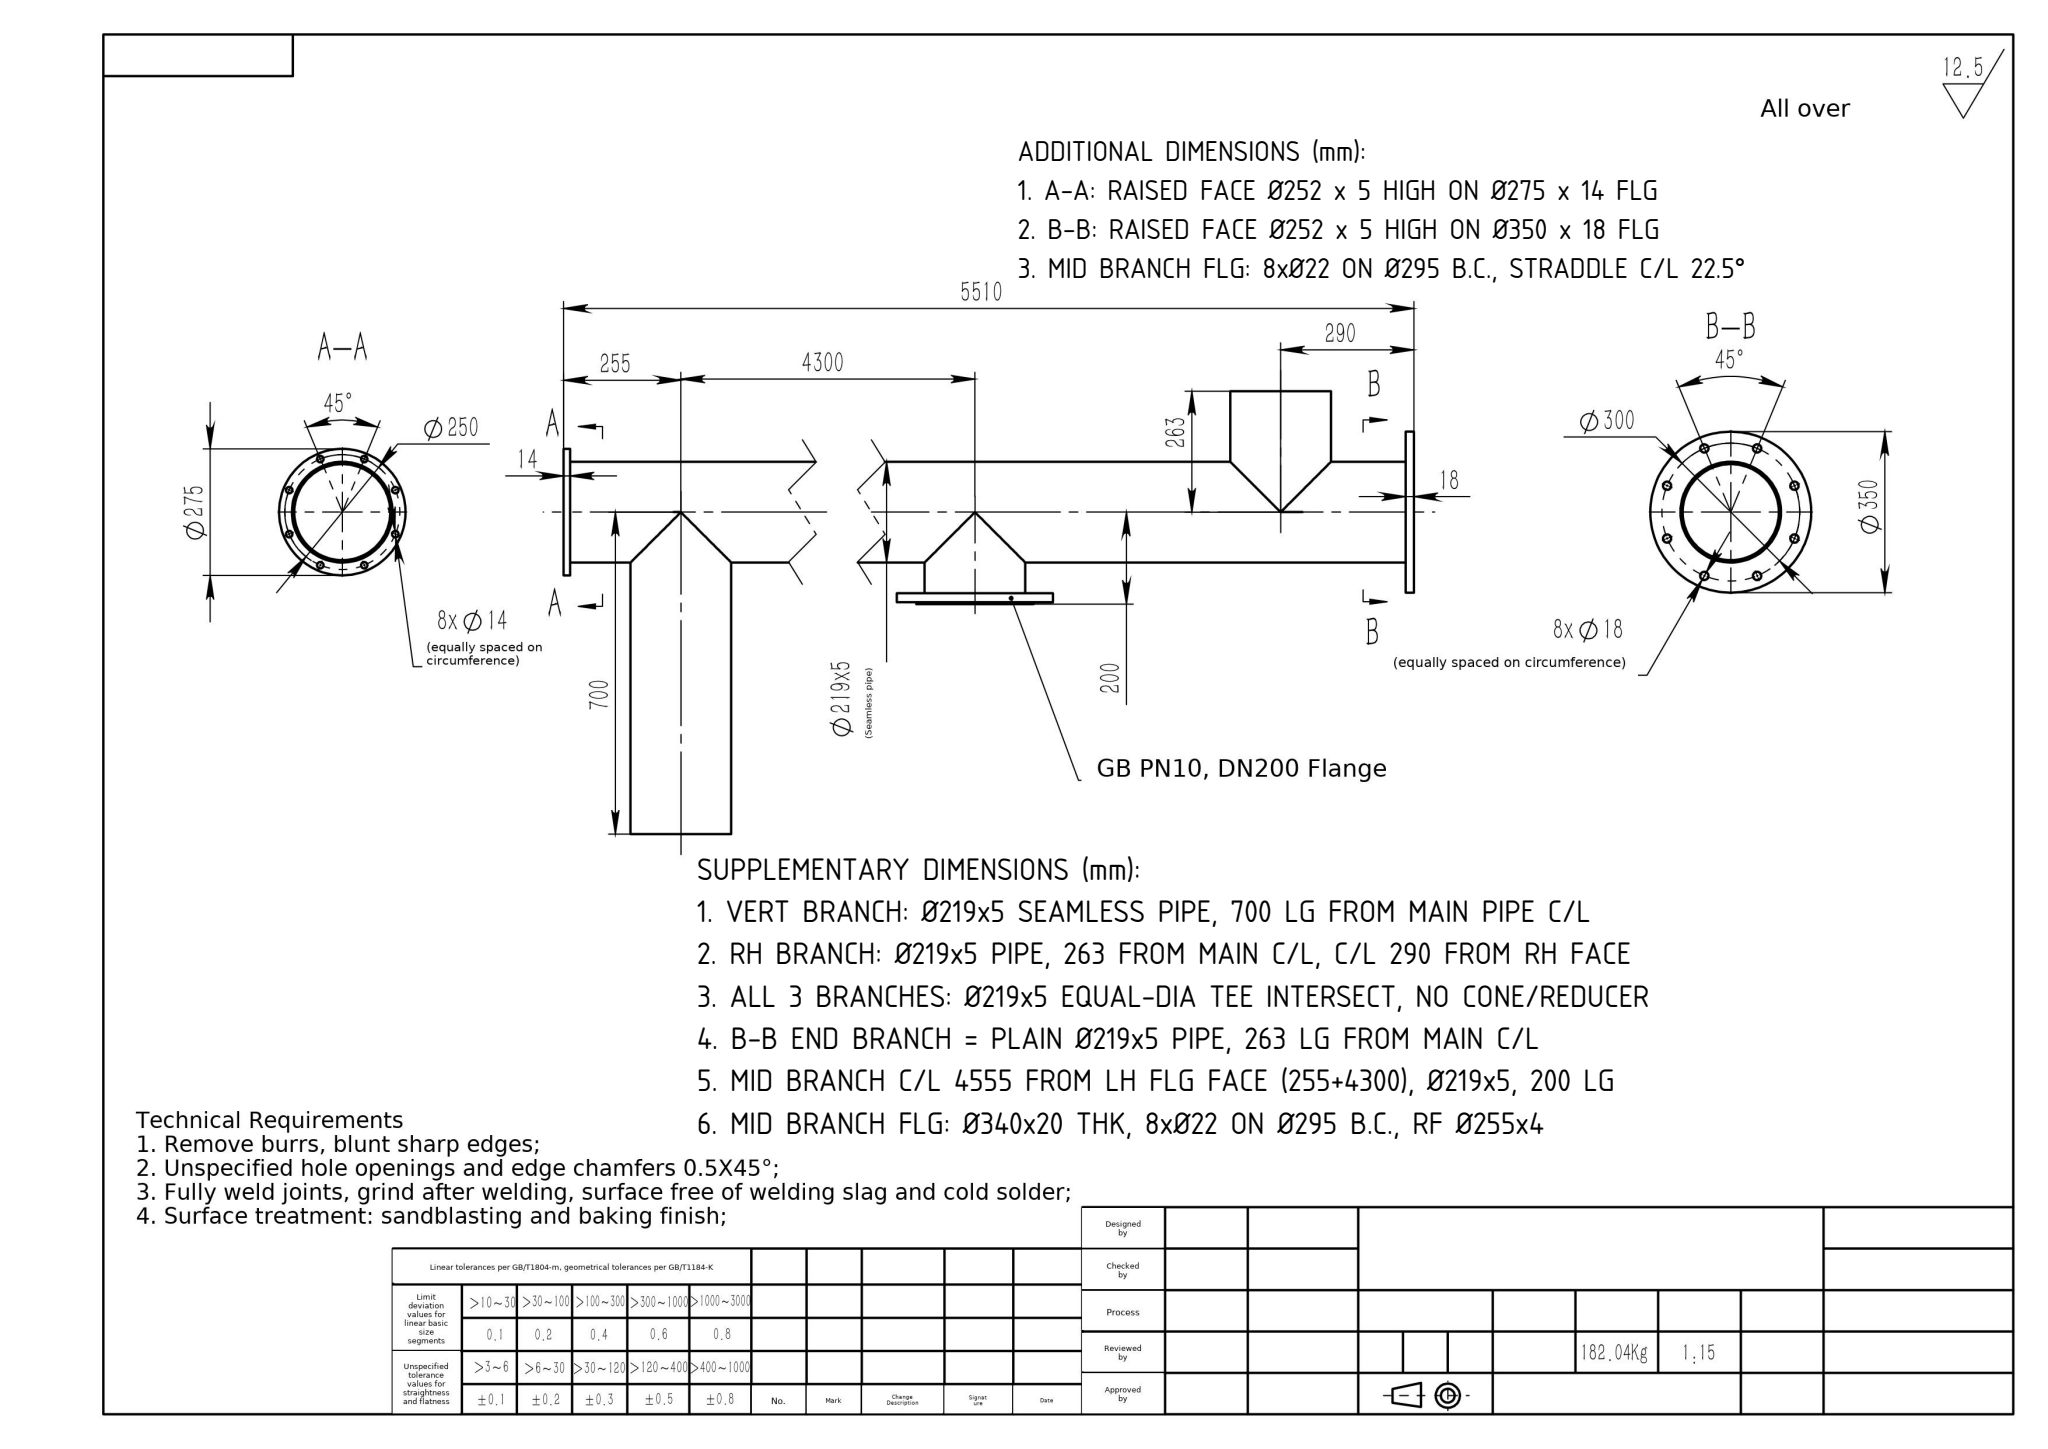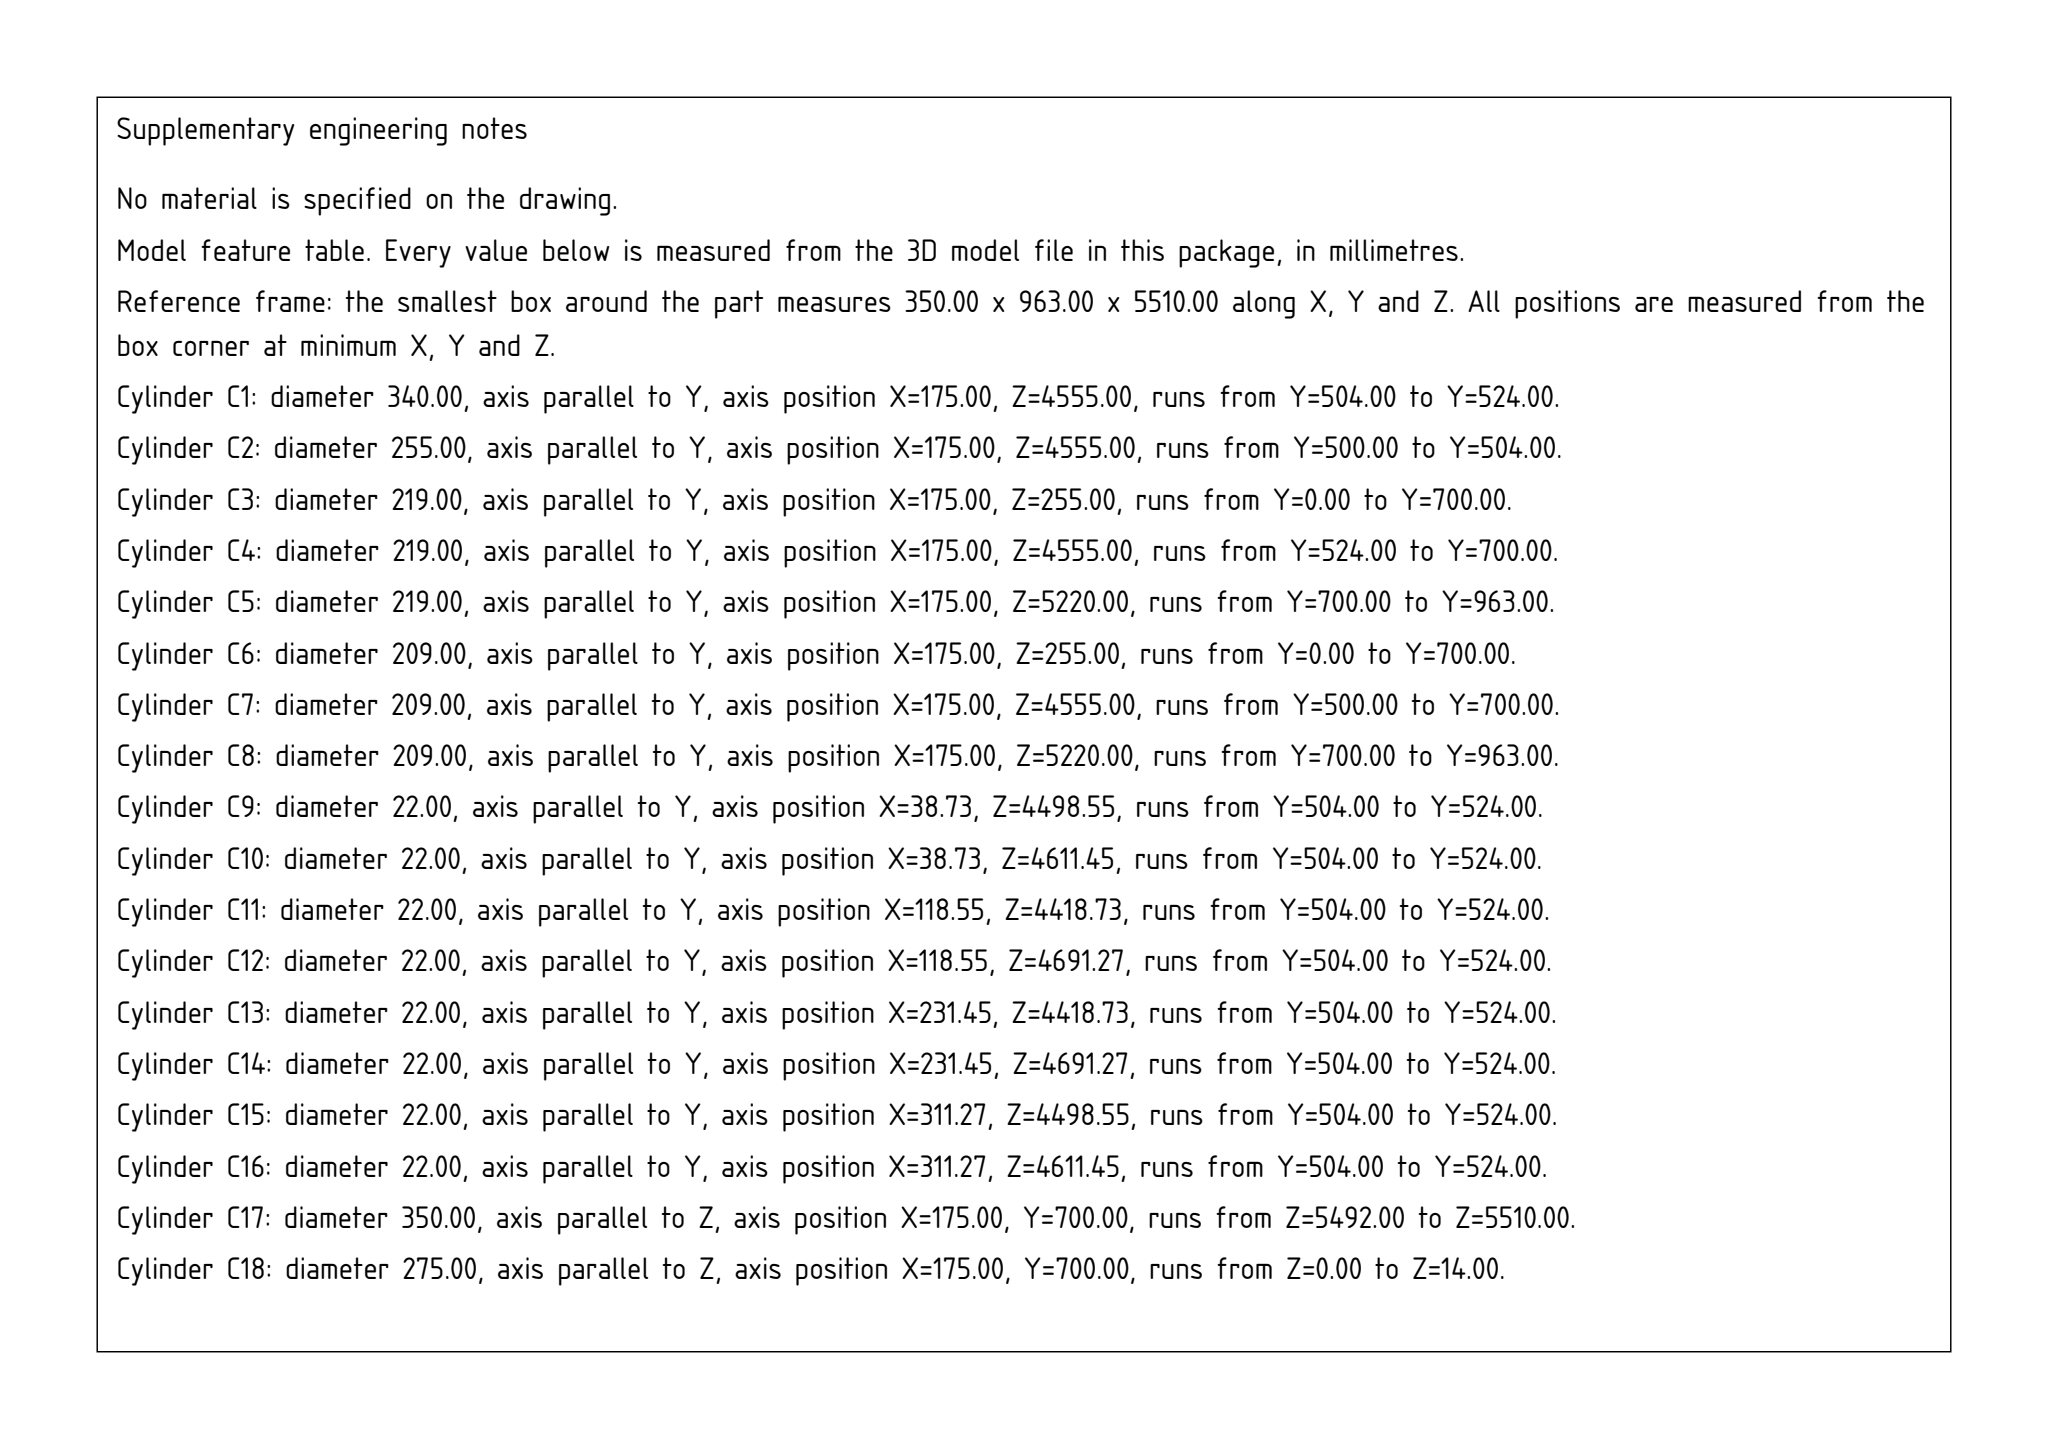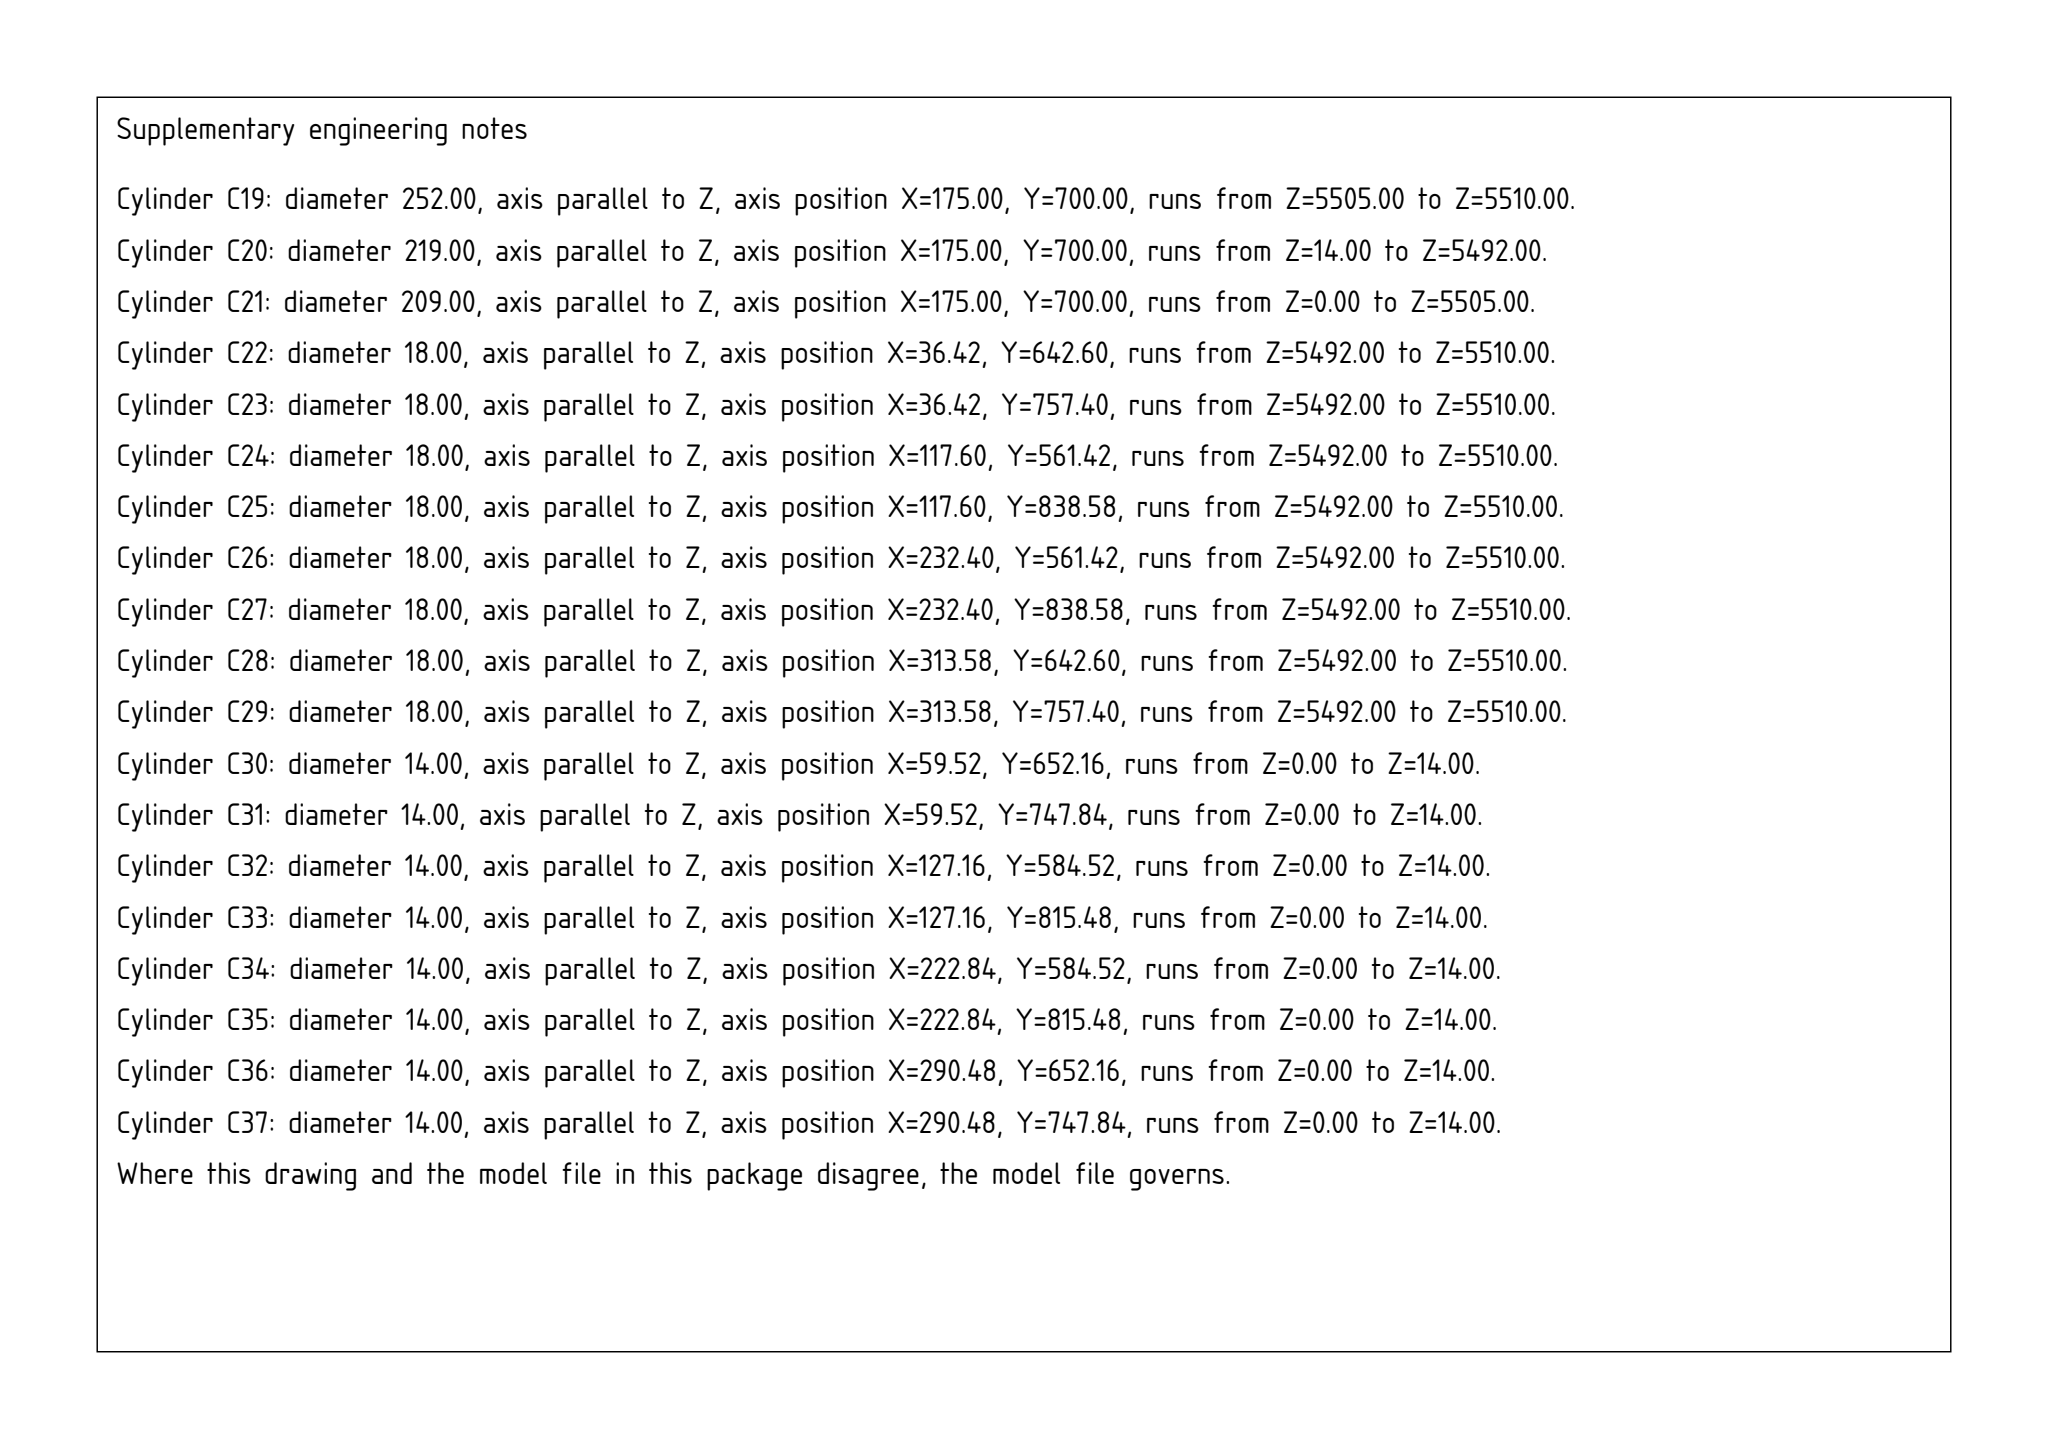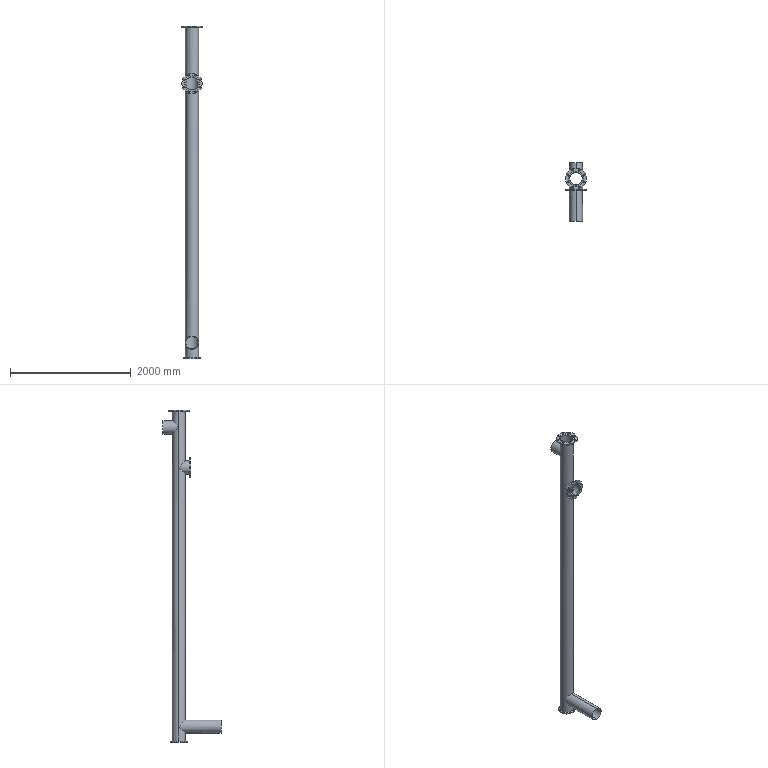Part | SolidWorks | mm | 1 solid | 90 faces | box 350 x 963 x 5510 mm | volume 23338668 mm3 | cylinder 80 | plane 10 | commonest cylinder face diameters 22 x16 14 x16 18 x16 209 x11 219 x11 340 x2 255 x2 275 x2